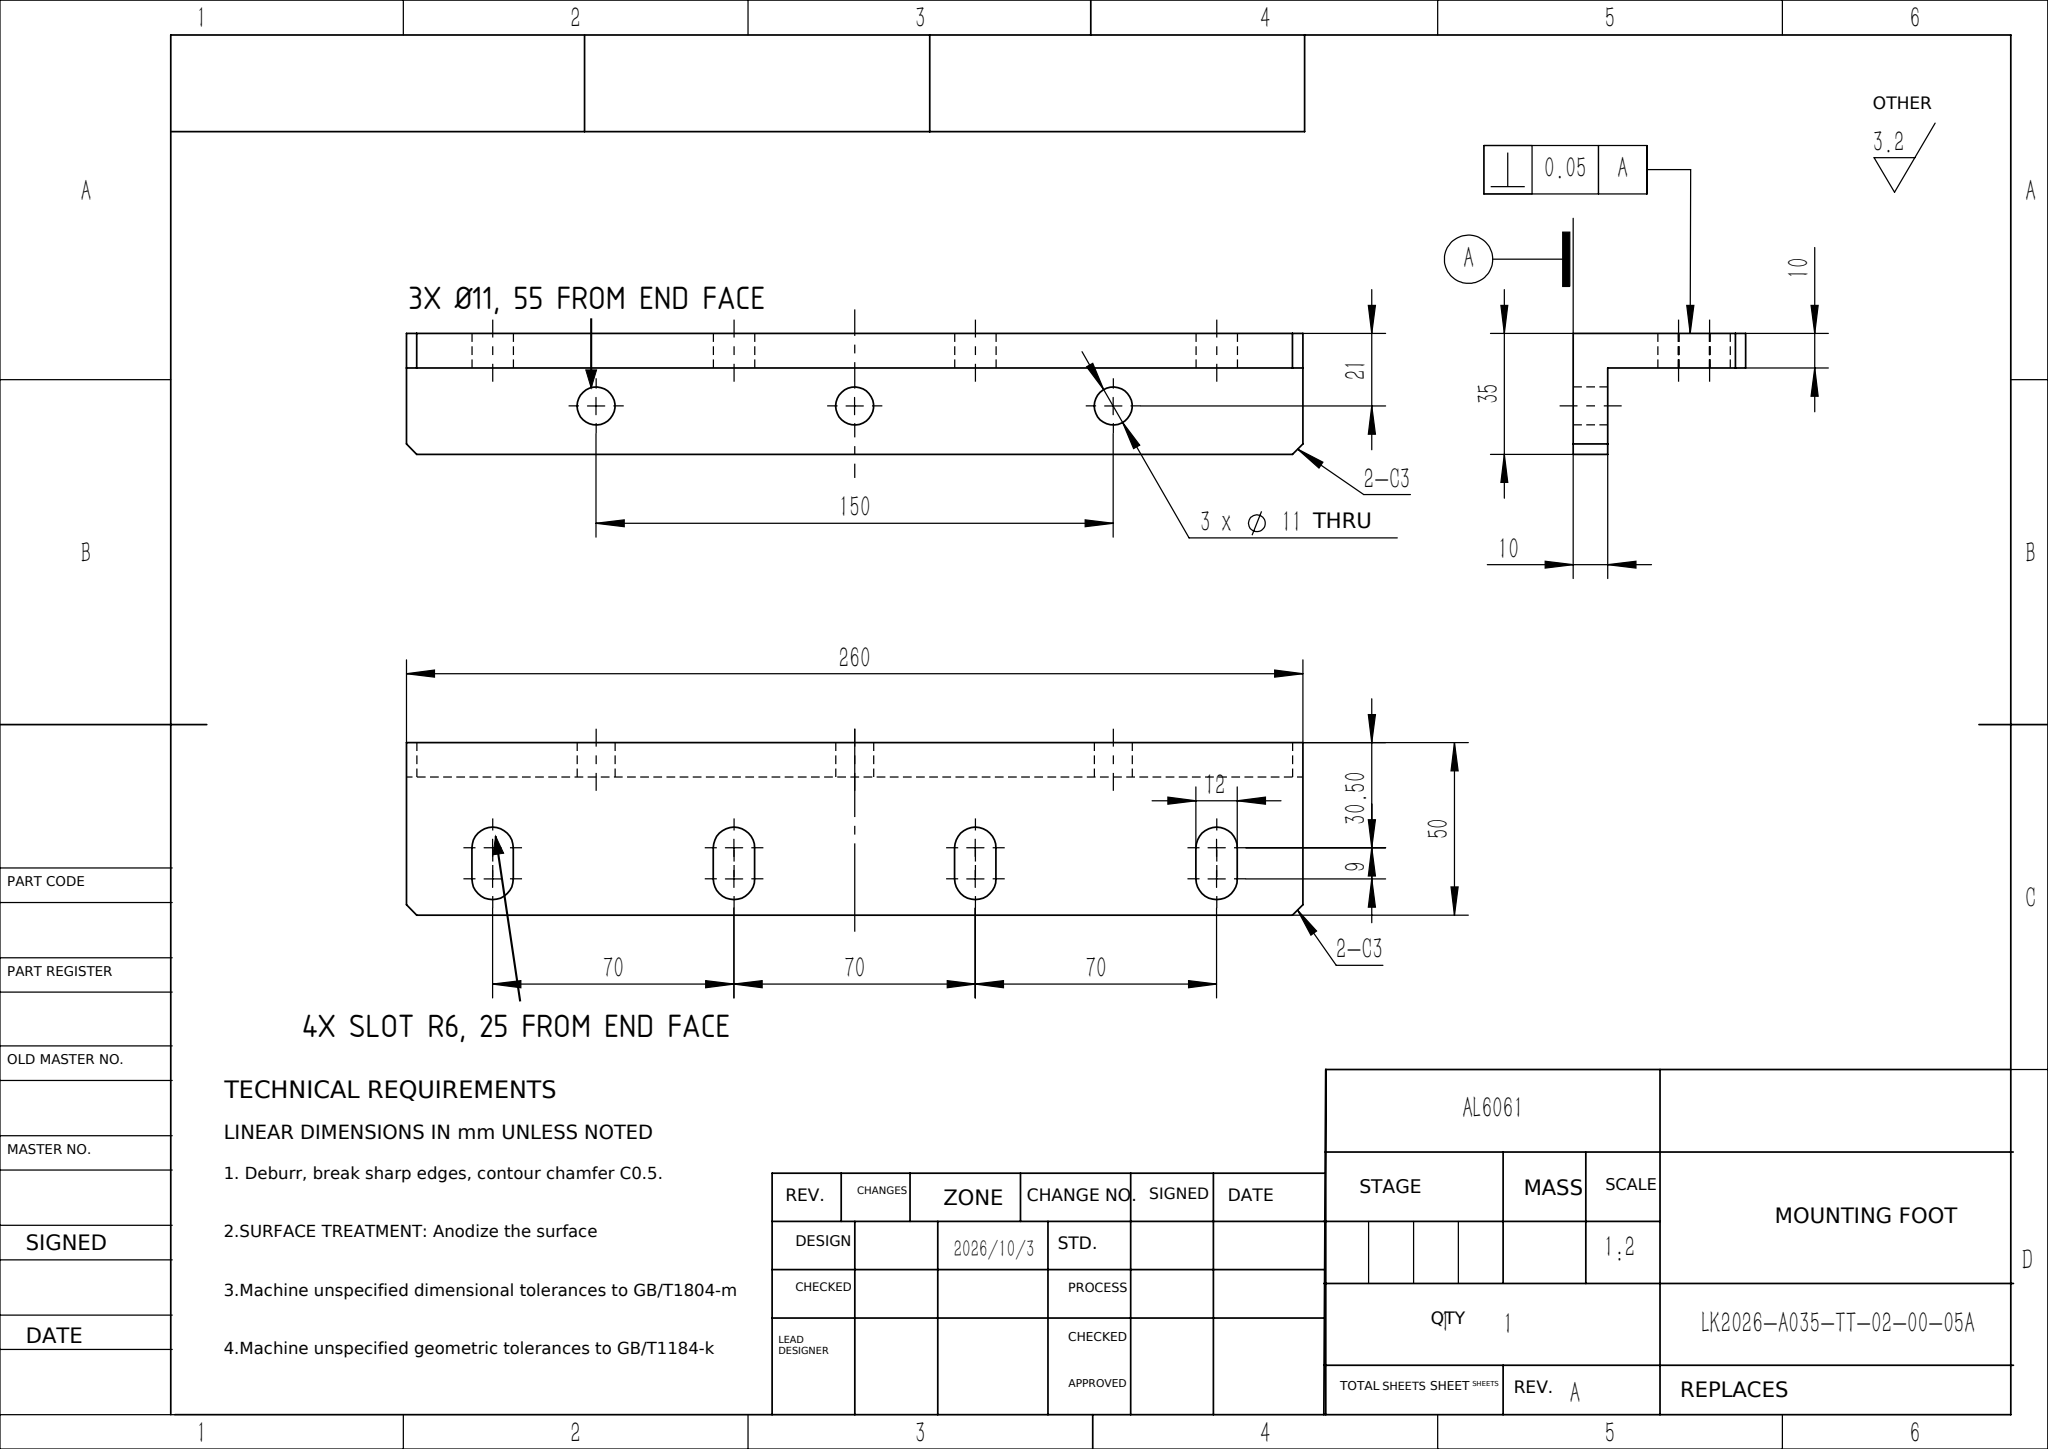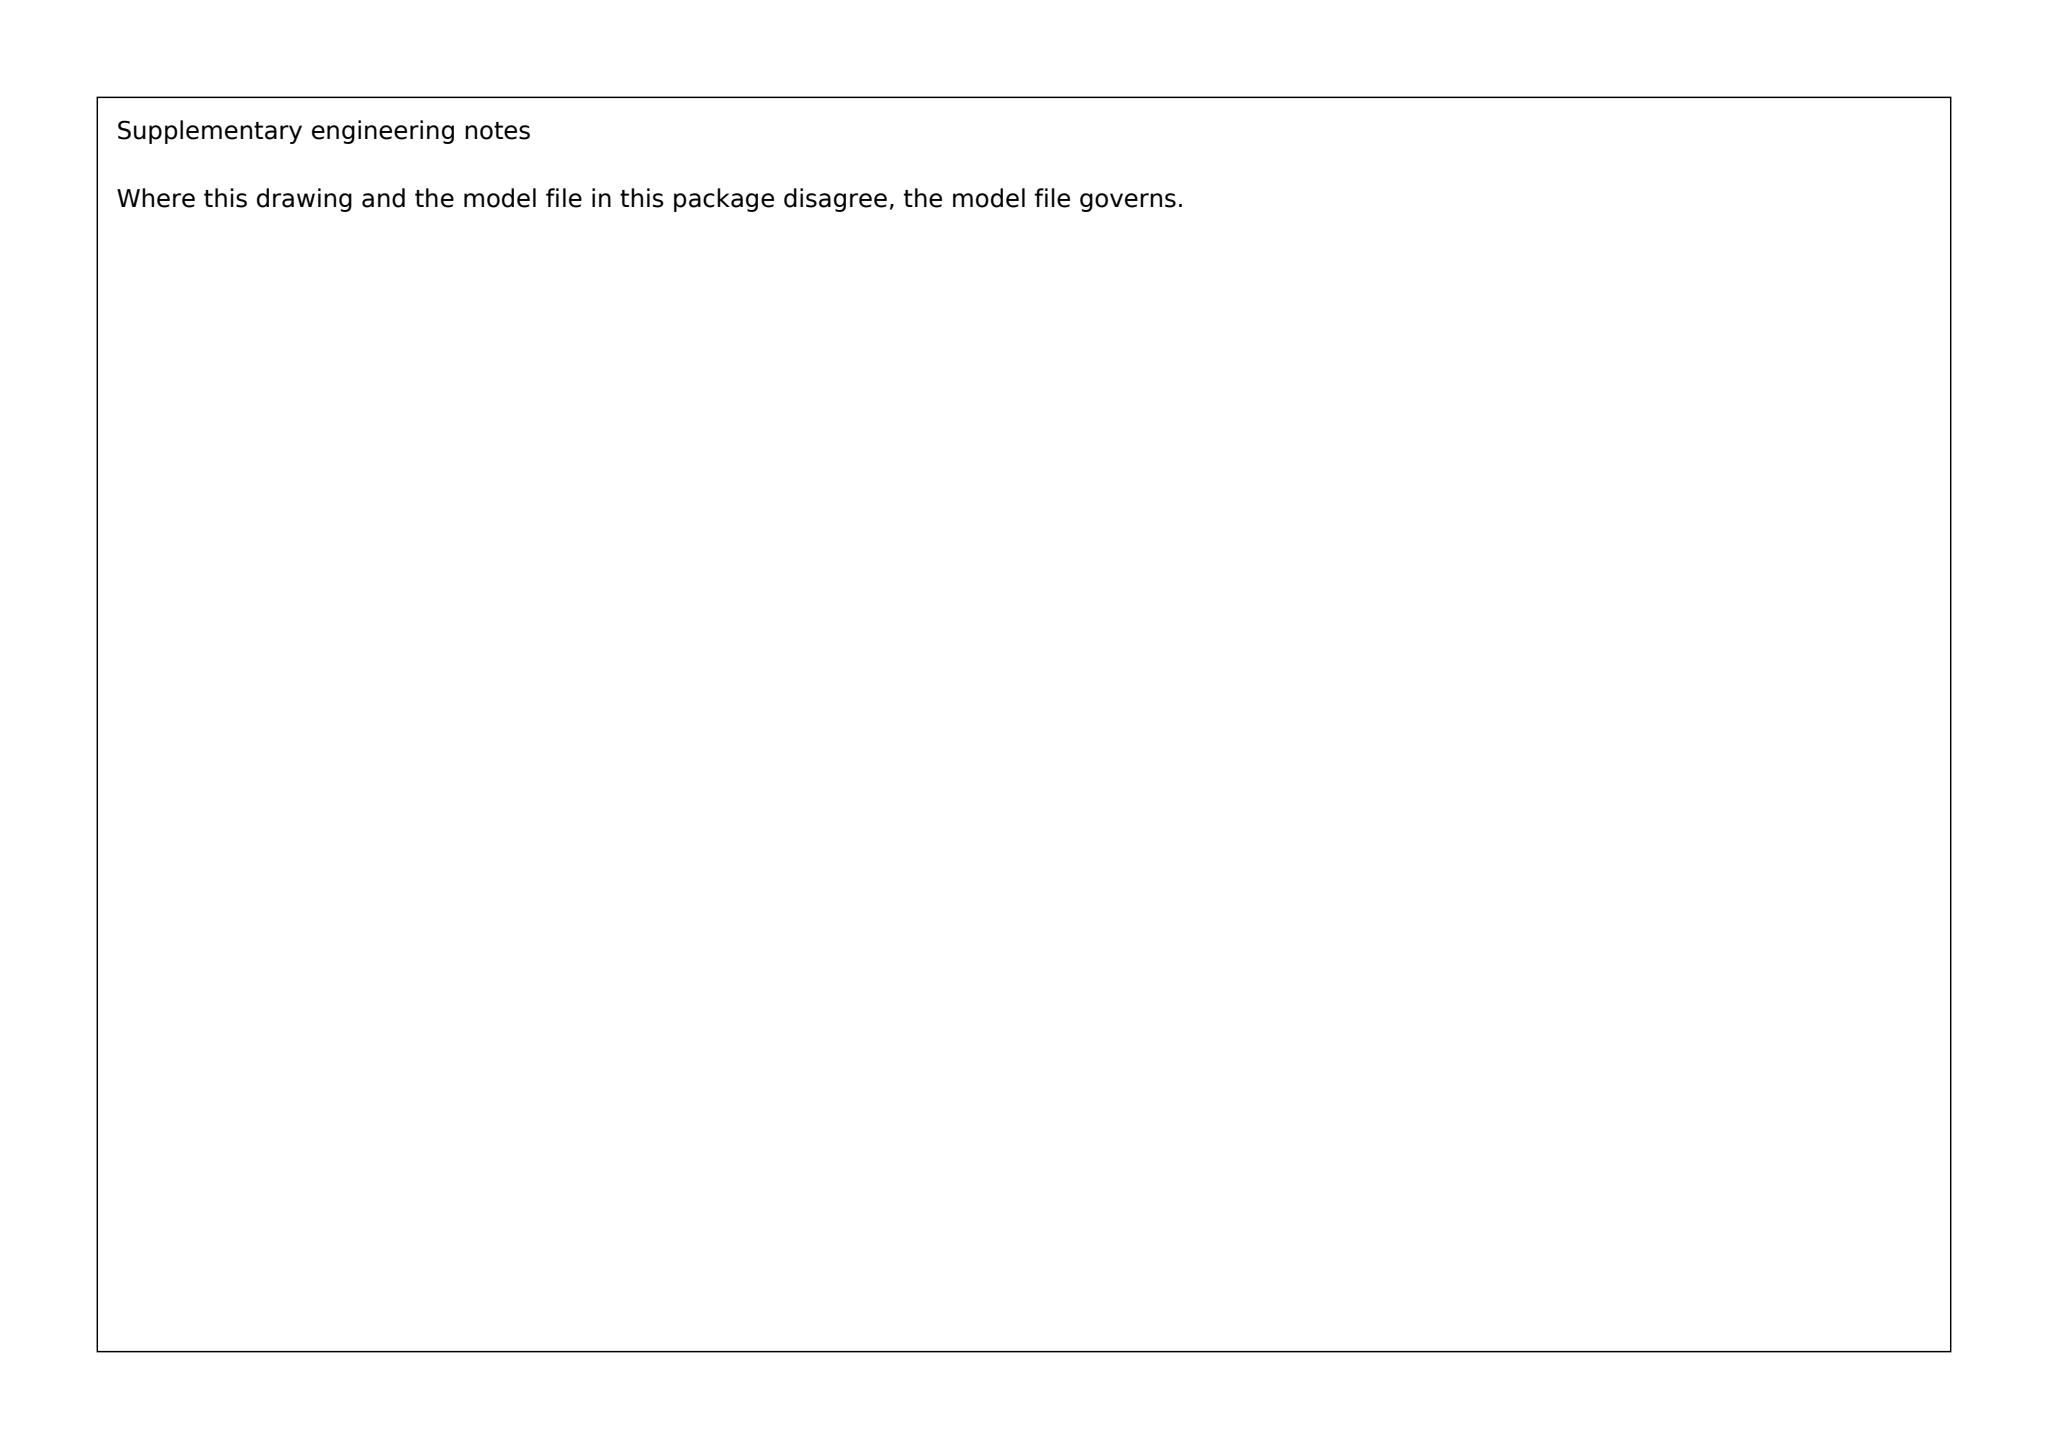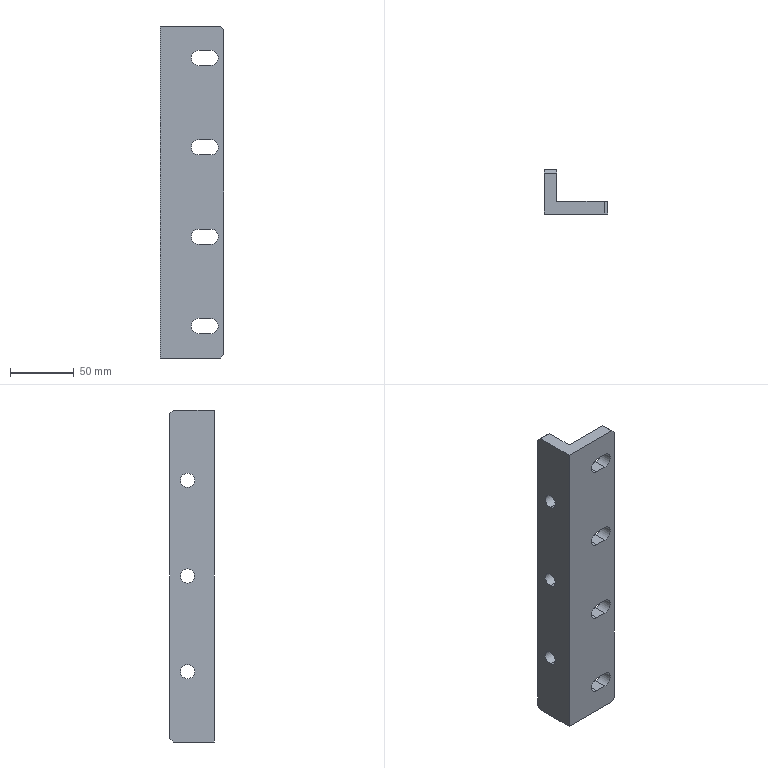Part | SolidWorks | mm | material AL6061 | 1 solid | 34 faces | box 50 x 35 x 260 mm | volume 183125 mm3 | plane 20 | cylinder 14 | commonest cylinder face diameters 12 x8 11 x6
Drawing notes:
3 x Ø11 THRU: 55 FROM END FACE, 75 PITCH | from the solid: Ø11 x-axis cyls at z=55,130,205; bbox z=0..260
4 x SLOT 12 W x 21 LG, R6 ENDS, CTRS 9 APART, 25 FROM END FACE | from the solid: Ø12 y-axis cyls paired x=30.5 & 39.5 at z=25,95,165,235; 9 apart => 21 oa, R6
build123d program:
from build123d import *

# Parameters (mm, degrees)
SKETCH1_W             = 50
SKETCH1_H             = 260
BOSS_EXTRUDE1_DEPTH   = 35
SKETCH2_W             = 40
SKETCH2_H             = 25
CUT_EXTRUDE1_DEPTH    = 268.067
CUT_EXTRUDE2_DEPTH    = 142.51
CUT_EXTRUDE3_DEPTH    = 142.51
CUT_EXTRUDE4_DEPTH    = 142.51
CUT_EXTRUDE5_DEPTH    = 144.614
M10_CLEARANCE_HOLE1_D = 11
CHAMFER1_SIZE         = 3


with BuildPart() as part:
    # Sketch1 → Boss-Extrude1 (new body)
    with BuildSketch(Plane(origin=(0, 35, 0), x_dir=(1, 0, 0), z_dir=(0, 1, 0))):
        with Locations((25, 0)):
            Rectangle(SKETCH1_W, SKETCH1_H)
    extrude(amount=-BOSS_EXTRUDE1_DEPTH)

    # Sketch2 → Cut-Extrude1 (cut, through all)
    with BuildSketch(Plane(origin=(0, 0, -130), x_dir=(-1, 0, 0), z_dir=(0, 0, -1))):
        with Locations((-30, 22.5)):
            Rectangle(SKETCH2_W, SKETCH2_H)
    extrude(amount=-CUT_EXTRUDE1_DEPTH, mode=Mode.SUBTRACT)

    # Sketch3 → Cut-Extrude2 (cut, through all)
    with BuildSketch(Plane(origin=(0, 10, 0), x_dir=(-1, 0, 0), z_dir=(0, 1, 0))):
        with BuildLine():
            Line((-30.5, -29), (-39.5, -29))
            ThreePointArc((-39.5, -29), (-45.5, -35), (-39.5, -41))
            Line((-39.5, -41), (-30.5, -41))
            ThreePointArc((-30.5, -41), (-24.5, -35), (-30.5, -29))
        make_face()
    extrude(amount=-CUT_EXTRUDE2_DEPTH, mode=Mode.SUBTRACT)

    # Sketch4 → Cut-Extrude3 (cut, through all)
    with BuildSketch(Plane(origin=(0, 10, 0), x_dir=(-1, 0, 0), z_dir=(0, 1, 0))):
        with BuildLine():
            Line((-30.5, 41), (-39.5, 41))
            ThreePointArc((-39.5, 41), (-45.5, 35), (-39.5, 29))
            Line((-39.5, 29), (-30.5, 29))
            ThreePointArc((-30.5, 29), (-24.5, 35), (-30.5, 41))
        make_face()
    extrude(amount=-CUT_EXTRUDE3_DEPTH, mode=Mode.SUBTRACT)

    # Sketch5 → Cut-Extrude4 (cut, through all)
    with BuildSketch(Plane(origin=(0, 10, 0), x_dir=(-1, 0, 0), z_dir=(0, 1, 0))):
        with BuildLine():
            Line((-30.5, -99), (-39.5, -99))
            ThreePointArc((-39.5, -99), (-45.5, -105), (-39.5, -111))
            Line((-39.5, -111), (-30.5, -111))
            ThreePointArc((-30.5, -111), (-24.5, -105), (-30.5, -99))
        make_face()
    extrude(amount=-CUT_EXTRUDE4_DEPTH, mode=Mode.SUBTRACT)

    # Sketch6 → Cut-Extrude5 (cut, through all)
    with BuildSketch(Plane.XZ):
        with BuildLine():
            Line((30.5, 99), (39.5, 99))
            ThreePointArc((39.5, 99), (45.5, 105), (39.5, 111))
            Line((39.5, 111), (30.5, 111))
            ThreePointArc((30.5, 111), (24.5, 105), (30.5, 99))
        make_face()
    extrude(amount=-CUT_EXTRUDE5_DEPTH, mode=Mode.SUBTRACT)

    # M10 Clearance Hole1 (through all)
    with Locations(Plane(origin=(10, 0, 0), x_dir=(0, 0, -1), z_dir=(1, 0, 0))):
        with Locations((75, 21), (0, 21), (-75, 21)):
            Hole(M10_CLEARANCE_HOLE1_D / 2)

    # Chamfer1
    chamfer1_edges = [part.edges().sort_by_distance(p)[0] for p in [
        (5, 35, -130),
        (5, 35, 130),
        (50, 5, -130),
        (50, 5, 130),
    ]]
    chamfer(chamfer1_edges, length=CHAMFER1_SIZE)


solid = part.part